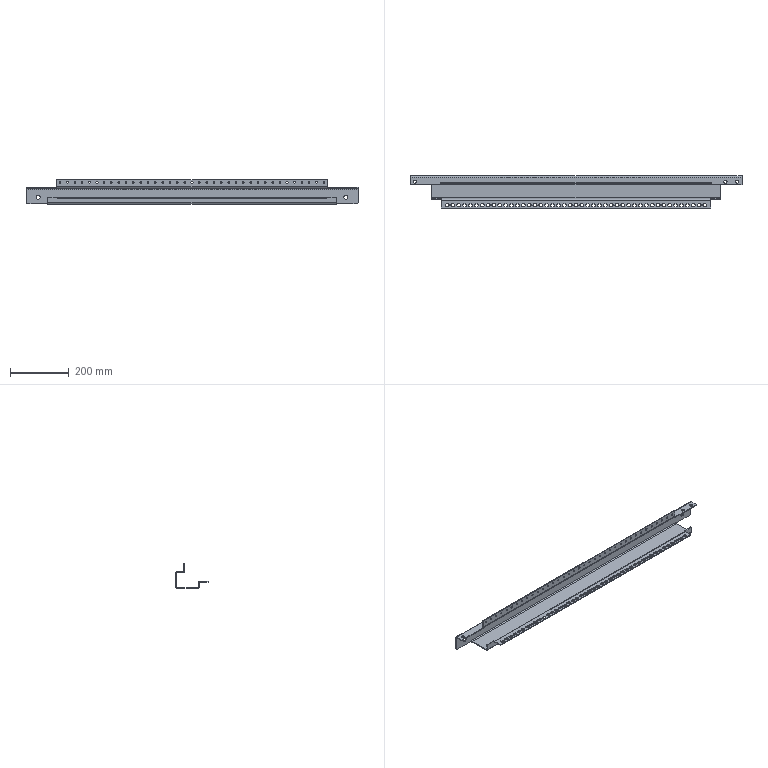Component | SolidWorks | SidePanelAssembly-1_HBSW.001.003SideTopBeam-1 | 1 solid | 334 faces | volume 689889 mm3 | cylinder 178 | plane 156 | commonest cylinder face diameters 9 x90 5.2 x68 11 x6 12 x5 6 x5 14 x4